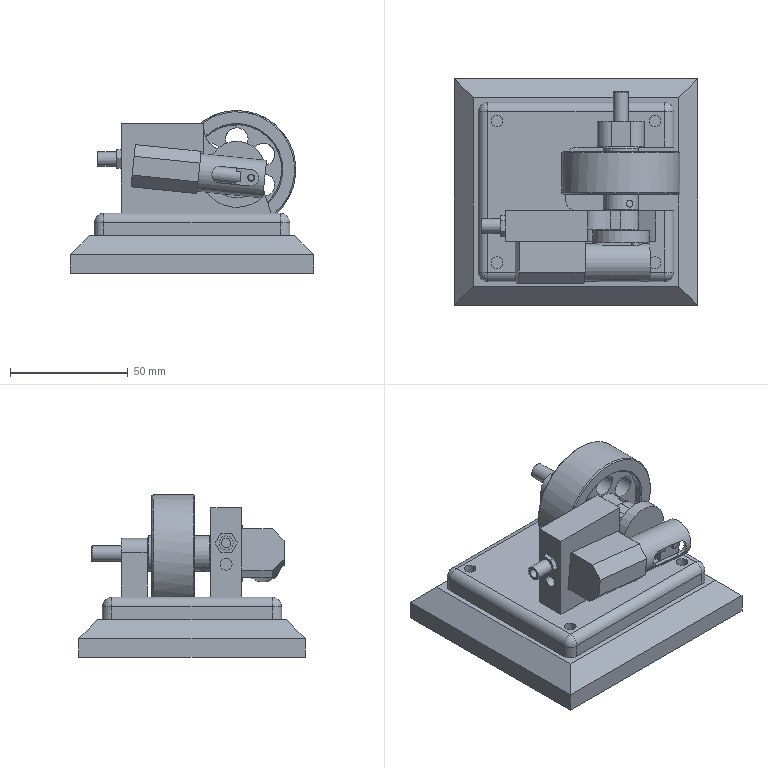Assembly | NX | mm | 9 component files | 9 solids | 178 faces | box 103 x 96 x 69 mm | volume 257007 mm3 | plane 90 | cylinder 71 | cone 11 | sphere 4 | torus 2 | commonest cylinder face diameters 4 x10 8 x9 6.5 x6 9.5 x6 3 x6 5 x5 13 x4 7 x4
Bill of materials:
unnamed part 1 | 1 |  | Straight hollow cylindrical tube with a hexagonal collar at roughly mid-length; through bore along the axis.
unnamed part 2 | 1 |  | Long slender cylindrical shaft with a disc-shaped flange near one end. A short, smaller-diameter pin sticks out of the far face of the disc, off the shaft axis, and a cross pin passes through the shaft near the flange.
unnamed part 3 | 1 |  | Turned pin with a large cylindrical head that has a small edge chamfer, a smaller-diameter cylindrical shank, and a flat rectangular tab at the far end with one small through hole.
unnamed part 4 | 1 |  | Rectangular block with one chamfered long edge. A hollow cylindrical tube sticks out from one end face, and a small solid cylindrical pin sticks out at right angles from a side of the block. The tube wall has an elongated slot with rounded ends.
unnamed part 5 | 1 |  | Rectangular block with both top corners rounded and one round through hole near the rounded end, like a clevis or lug block.
unnamed part 6 | 1 |  | Wheel- or pulley-like disc with a wide cylindrical rim, a recessed web holding six circular lightening holes evenly spaced on a circle, and a central hub that sticks out from both faces. The hub has an axial bore and a small radial hole.
unnamed part 7 | 1 |  | Thick, mostly rectangular plate with an irregular profile on one end: a concave arc cutout, a rounded lobe holding a large through hole, and an angled edge. The lobe area is stepped to a different thickness from the main body. It has one medium through hole and two small holes in the main body.
unnamed part 8 | 1 |  | Square flat plate with a chamfered (beveled) edge all the way around the top face; no holes or other features.
unnamed part 9 | 1 |  | Rectangular plate with rounded corners and filleted top edges. A U-shaped slot with rounded inner corners is open on one side. It has four larger corner holes and four smaller through holes.
Mates:
1. fix | base 1 component
2. touch align | base_plate 1 face | base 1 face
3. center | base_plate 1 face | base_plate 1 face | base 1 face | base 1 face
4. center | base_plate 1 face | base_plate 1 face | base 1 face | base 1 face
5. concentric | base_plate 1 edge | bracket 1 arc
6. parallel | bracket 1 face | base_plate 1 face
7. concentric | base_plate 1 edge | small_bracket 1 arc
8. parallel | small_bracket 1 face | base_plate 1 face
9. concentric | bracket 1 edge | pipe 1 arc
10. parallel | pipe 1 face | bracket 1 face
11. touch align | crankshaft 1 face | flywheel 1 face
12. touch align | crankshaft 1 face | flywheel 1 face
13. touch align | crankshaft 1 face | small_bracket 1 face
14. touch align | flywheel 1 face | small_bracket 1 face
15. touch align | piston_cylinder 1 face | bracket 1 face
16. touch align | piston_cylinder 1 face | bracket 1 face
17. touch align | piston 1 face | piston_cylinder 1 face
18. touch align | piston 1 face | crankshaft 1 face